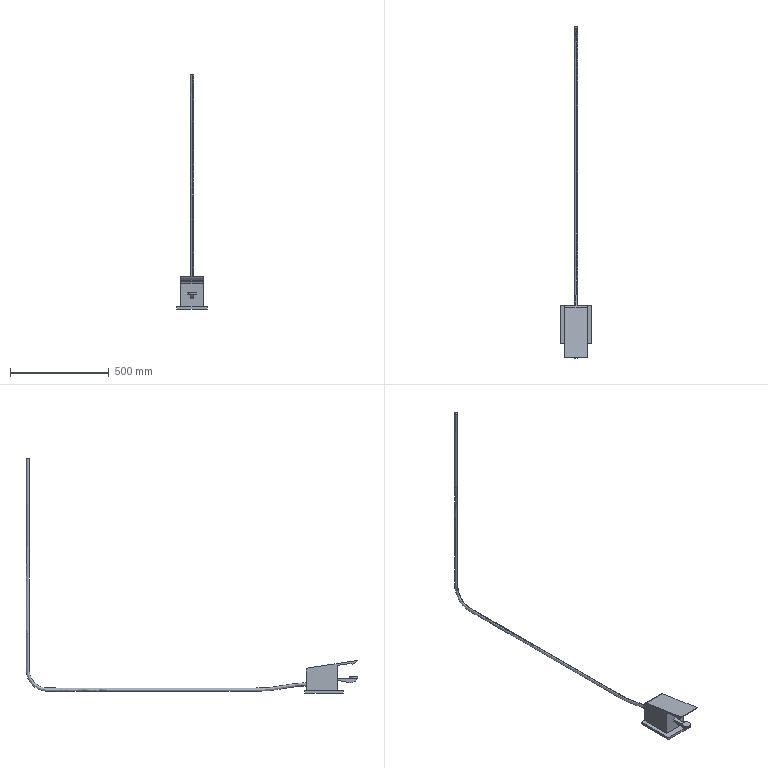Component | SolidWorks | FootSwitch-2 | 1 solid | 31 faces | volume 3348846 mm3 | plane 23 | cylinder 6 | spline 2 | commonest cylinder face diameters 43 x2 20 x2 55.805 x1 82 x1